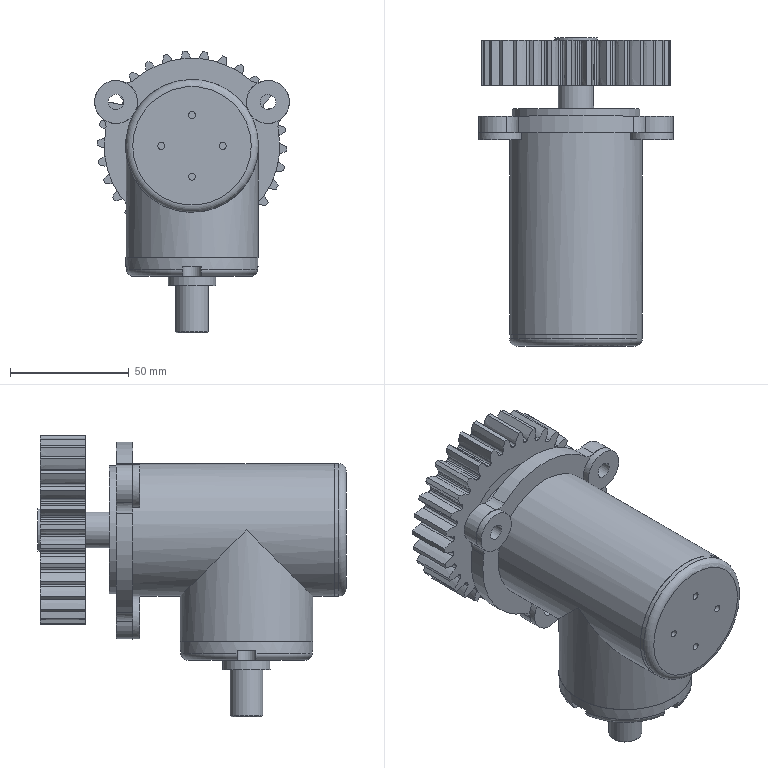Assembly | NX | mm | 11 component files | 11 solids | 391 faces | box 82.19 x 130 x 118.82 mm | volume 306073 mm3 | other 150 | cylinder 122 | plane 97 | spline 10 | cone 7 | torus 5 | commonest cylinder face diameters 68.75 x30 4 x7 12 x6 10 x6 4.5 x5 15 x4 22 x4 56 x4
Bill of materials:
unnamed part 1 | 1 |  | Plug-like part: a thin round flange head with a rounded outer edge, and a shorter cylindrical body with external threads standing up from one face. There is a plain neck between the flange and the threads.
unnamed part 2 | 1 |  | Straight-toothed spur gear: a flat disc with roughly 30 teeth around the rim, a central bore with one keyway, and a recessed ring-shaped pocket on one face around a raised hub.
unnamed part 3 | 1 |  | Flanged hub: a round flange with four evenly spaced through holes, and a raised cylindrical boss with a large central through bore. The underside has a rounded edge and small notches or slots cut into the rim.
unnamed part 4 | 1 |  | Hollow T-shaped body: a main cylindrical tube with internal threads at its open end, a cylindrical branch joining it at right angles, and a flange at the other end with two lugs (ears) that each have a hole. The flange face has a smaller central opening and a ring-shaped step or groove.
unnamed part 5 | 1 |  | Flanged sleeve: a thick-walled cylindrical tube with a through bore and an outer flange set a short distance from one end. A shallow groove runs around the outside near the opposite end.
unnamed part 6 | 1 |  | Thin flat ring disc (washer-like): a large outer diameter, a small central round hole and uniform thickness.
unnamed part 7 | 1 |  | Solid stepped round shaft with several diameters along its axis: a short largest-diameter collar, a long middle section, and smaller sections at each end.
unnamed part 8 | 1 |  | Teardrop-shaped lever or clevis block: a large through bore at the wide rounded end, a small cross hole at the tapered end, and a rectangular slot cut through the tapered end that forms two prongs.
unnamed part 9 | 2 |  | Plain thick-walled cylindrical ring (spacer- or bushing-like) with a uniform through bore and flat end faces.
unnamed part 10 | 1 |  | Cylindrical pin with a flat tang at one end. The tang has a rounded tip and a cross hole, and a small step sits between the tang and the cylindrical shank.
Mates:
1. fix | 1 1 component
2. touch align | 5 1 face | 3 1 face
3. center | 3 1 face | 3 1 face | 5 1 face | 5 1 face
4. touch align | 6 1 face | 3 1 face
5. touch align | 6 1 face | 3 1 face
6. touch align | 6 1 face | 1 1 face
7. touch align | 5 1 face | 1 1 face
8. concentric | 1 1 edge | 9 1 edge
9. concentric | 1 1 edge | 9 1 edge
10. concentric | 9 1 arc | 7 1 edge
11. parallel | 4 1 face | 6 1 face
12. touch align | 4 1 face | 6 1 face
13. touch align | 6 1 face | 4 1 face
14. concentric | 11 1 arc | 4 1 arc
15. concentric | 6 1 edge | 8 2 arc
16. concentric | 6 1 edge | 8 1 arc
17. concentric | 1 1 edge | 10 1 edge